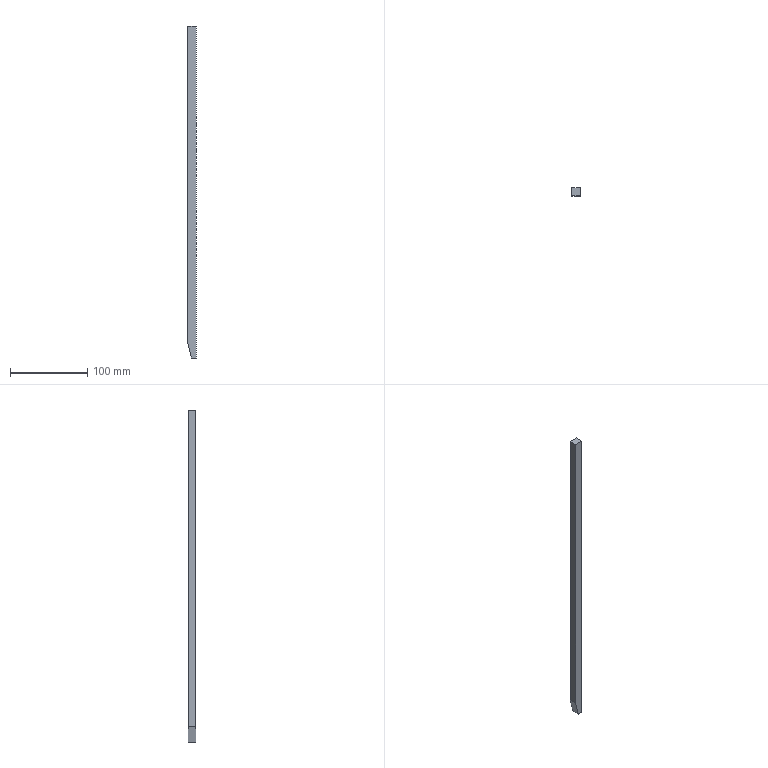Component | SolidWorks | CHEN123-AA-19-1 | 1 solid | 7 faces | box 11.5 x 10 x 430 mm | volume 48950 mm3 | plane 7
build123d program:
from build123d import *

# Parameters (mm, degrees)
SKETCH1_W           = 430
SKETCH1_H           = 11.5
BOSS_EXTRUDE1_DEPTH = 10
CHAMFER1_SIZE       = 20
CHAMFER1_SIZE2      = 5


with BuildPart() as part:
    # Sketch1 → Boss-Extrude1 (new body)
    with BuildSketch(Plane.XY):
        Rectangle(SKETCH1_W, SKETCH1_H)
    extrude(amount=BOSS_EXTRUDE1_DEPTH)

    # Chamfer1
    chamfer1_edges = [part.edges().sort_by_distance(p)[0] for p in [
        (-215, -5.75, 5),
    ]]
    chamfer1_side = [part.faces().sort_by_distance(p)[0] for p in [
        (0, -5.75, 5),
    ]]
    chamfer(chamfer1_edges, length=CHAMFER1_SIZE, length2=CHAMFER1_SIZE2, reference=chamfer1_side[0])


solid = part.part

# Placed as in the assembly
solid = solid.moved(Location((22.25, 34.001, -205), (-90, 0, -90)))
STEP:
#1=COLOUR_RGB('',0.7922,0.8196,0.9333);
#2=FILL_AREA_STYLE_COLOUR('',#1);
#3=FILL_AREA_STYLE('',(#2));
#4=SURFACE_STYLE_FILL_AREA(#3);
#5=SURFACE_SIDE_STYLE('',(#4));
#6=SURFACE_STYLE_USAGE(.BOTH.,#5);
#7=PRESENTATION_STYLE_ASSIGNMENT((#6));
#8=CARTESIAN_POINT('',(0.6496,1.339,0.3937));
#9=VERTEX_POINT('',#8);
#10=CARTESIAN_POINT('',(1.102,1.339,0.3937));
#11=VERTEX_POINT('',#10);
#12=CARTESIAN_POINT('',(0.6496,1.339,0.3937));
#13=DIRECTION('',(1.,-0.,-0.));
#14=VECTOR('',#13,39.37);
#15=LINE('',#12,#14);
#16=EDGE_CURVE('',#9,#11,#15,.T.);
#17=ORIENTED_EDGE('',*,*,#16,.T.);
#18=CARTESIAN_POINT('',(1.102,1.732,0.3937));
#19=VERTEX_POINT('',#18);
#20=CARTESIAN_POINT('',(1.102,1.732,0.3937));
#21=DIRECTION('',(-0.,-1.,0.));
#22=VECTOR('',#21,39.37);
#23=LINE('',#20,#22);
#24=EDGE_CURVE('',#19,#11,#23,.T.);
#25=ORIENTED_EDGE('',*,*,#24,.F.);
#26=CARTESIAN_POINT('',(0.6496,1.732,0.3937));
#27=VERTEX_POINT('',#26);
#28=CARTESIAN_POINT('',(0.6496,1.732,0.3937));
#29=DIRECTION('',(1.,-0.,-0.));
#30=VECTOR('',#29,39.37);
#31=LINE('',#28,#30);
#32=EDGE_CURVE('',#27,#19,#31,.T.);
#33=ORIENTED_EDGE('',*,*,#32,.F.);
#34=CARTESIAN_POINT('',(0.6496,1.732,0.3937));
#35=DIRECTION('',(-0.,-1.,0.));
#36=VECTOR('',#35,39.37);
#37=LINE('',#34,#36);
#38=EDGE_CURVE('',#27,#9,#37,.T.);
#39=ORIENTED_EDGE('',*,*,#38,.T.);
#40=EDGE_LOOP('',(#17,#25,#33,#39));
#41=FACE_OUTER_BOUND('',#40,.T.);
#42=CARTESIAN_POINT('',(0.6496,1.732,0.3937));
#43=DIRECTION('',(-0.,-0.,-1.));
#44=DIRECTION('',(0.,1.,-0.));
#45=AXIS2_PLACEMENT_3D('',#42,#43,#44);
#46=PLANE('',#45);
#47=ADVANCED_FACE('',(#41),#46,.F.);
#48=CARTESIAN_POINT('',(1.102,1.339,-16.535));
#49=VERTEX_POINT('',#48);
#50=CARTESIAN_POINT('',(1.102,1.339,-16.535));
#51=DIRECTION('',(-0.,0.,-1.));
#52=VECTOR('',#51,39.37);
#53=LINE('',#50,#52);
#54=EDGE_CURVE('',#11,#49,#53,.T.);
#55=ORIENTED_EDGE('',*,*,#54,.T.);
#56=CARTESIAN_POINT('',(1.102,1.732,-16.535));
#57=VERTEX_POINT('',#56);
#58=CARTESIAN_POINT('',(1.102,1.732,-16.535));
#59=DIRECTION('',(-0.,-1.,0.));
#60=VECTOR('',#59,39.37);
#61=LINE('',#58,#60);
#62=EDGE_CURVE('',#57,#49,#61,.T.);
#63=ORIENTED_EDGE('',*,*,#62,.F.);
#64=CARTESIAN_POINT('',(1.102,1.732,-16.535));
#65=DIRECTION('',(-0.,0.,-1.));
#66=VECTOR('',#65,39.37);
#67=LINE('',#64,#66);
#68=EDGE_CURVE('',#19,#57,#67,.T.);
#69=ORIENTED_EDGE('',*,*,#68,.F.);
#70=ORIENTED_EDGE('',*,*,#24,.T.);
#71=EDGE_LOOP('',(#55,#63,#69,#70));
#72=FACE_OUTER_BOUND('',#71,.T.);
#73=CARTESIAN_POINT('',(1.102,1.732,-16.535));
#74=DIRECTION('',(-1.,0.,0.));
#75=DIRECTION('',(-0.,-1.,0.));
#76=AXIS2_PLACEMENT_3D('',#73,#74,#75);
#77=PLANE('',#76);
#78=ADVANCED_FACE('',(#72),#77,.F.);
#79=CARTESIAN_POINT('',(0.8464,1.339,-16.535));
#80=VERTEX_POINT('',#79);
#81=CARTESIAN_POINT('',(0.6496,1.339,-16.535));
#82=DIRECTION('',(-1.,0.,0.));
#83=VECTOR('',#82,39.37);
#84=LINE('',#81,#83);
#85=EDGE_CURVE('',#49,#80,#84,.T.);
#86=ORIENTED_EDGE('',*,*,#85,.T.);
#87=CARTESIAN_POINT('',(0.8464,1.732,-16.535));
#88=VERTEX_POINT('',#87);
#89=CARTESIAN_POINT('',(0.8464,1.732,-16.535));
#90=DIRECTION('',(0.,1.,-0.));
#91=VECTOR('',#90,39.37);
#92=LINE('',#89,#91);
#93=EDGE_CURVE('',#80,#88,#92,.T.);
#94=ORIENTED_EDGE('',*,*,#93,.T.);
#95=CARTESIAN_POINT('',(0.6496,1.732,-16.535));
#96=DIRECTION('',(-1.,0.,0.));
#97=VECTOR('',#96,39.37);
#98=LINE('',#95,#97);
#99=EDGE_CURVE('',#57,#88,#98,.T.);
#100=ORIENTED_EDGE('',*,*,#99,.F.);
#101=ORIENTED_EDGE('',*,*,#62,.T.);
#102=EDGE_LOOP('',(#86,#94,#100,#101));
#103=FACE_OUTER_BOUND('',#102,.T.);
#104=CARTESIAN_POINT('',(0.6496,1.732,-16.535));
#105=DIRECTION('',(0.,0.,1.));
#106=DIRECTION('',(-0.,-1.,0.));
#107=AXIS2_PLACEMENT_3D('',#104,#105,#106);
#108=PLANE('',#107);
#109=ADVANCED_FACE('',(#103),#108,.F.);
#110=CARTESIAN_POINT('',(0.6496,1.732,-15.748));
#111=VERTEX_POINT('',#110);
#112=CARTESIAN_POINT('',(0.6496,1.732,-16.535));
#113=DIRECTION('',(0.,-0.,1.));
#114=VECTOR('',#113,39.37);
#115=LINE('',#112,#114);
#116=EDGE_CURVE('',#111,#27,#115,.T.);
#117=ORIENTED_EDGE('',*,*,#116,.F.);
#118=CARTESIAN_POINT('',(0.6496,1.339,-15.748));
#119=VERTEX_POINT('',#118);
#120=CARTESIAN_POINT('',(0.6496,1.732,-15.748));
#121=DIRECTION('',(-0.,-1.,0.));
#122=VECTOR('',#121,39.37);
#123=LINE('',#120,#122);
#124=EDGE_CURVE('',#111,#119,#123,.T.);
#125=ORIENTED_EDGE('',*,*,#124,.T.);
#126=CARTESIAN_POINT('',(0.6496,1.339,-16.535));
#127=DIRECTION('',(0.,-0.,1.));
#128=VECTOR('',#127,39.37);
#129=LINE('',#126,#128);
#130=EDGE_CURVE('',#119,#9,#129,.T.);
#131=ORIENTED_EDGE('',*,*,#130,.T.);
#132=ORIENTED_EDGE('',*,*,#38,.F.);
#133=EDGE_LOOP('',(#117,#125,#131,#132));
#134=FACE_OUTER_BOUND('',#133,.T.);
#135=CARTESIAN_POINT('',(0.6496,1.732,-16.535));
#136=DIRECTION('',(1.,-0.,-0.));
#137=DIRECTION('',(0.,1.,-0.));
#138=AXIS2_PLACEMENT_3D('',#135,#136,#137);
#139=PLANE('',#138);
#140=ADVANCED_FACE('',(#134),#139,.F.);
#141=ORIENTED_EDGE('',*,*,#99,.T.);
#142=CARTESIAN_POINT('',(0.6496,1.732,-15.748));
#143=DIRECTION('',(-0.2425,-0.,0.9701));
#144=VECTOR('',#143,39.37);
#145=LINE('',#142,#144);
#146=EDGE_CURVE('',#88,#111,#145,.T.);
#147=ORIENTED_EDGE('',*,*,#146,.T.);
#148=ORIENTED_EDGE('',*,*,#116,.T.);
#149=ORIENTED_EDGE('',*,*,#32,.T.);
#150=ORIENTED_EDGE('',*,*,#68,.T.);
#151=EDGE_LOOP('',(#141,#147,#148,#149,#150));
#152=FACE_OUTER_BOUND('',#151,.T.);
#153=CARTESIAN_POINT('',(0.876,1.732,-8.071));
#154=DIRECTION('',(-0.,-1.,-0.));
#155=DIRECTION('',(-0.,0.,-1.));
#156=AXIS2_PLACEMENT_3D('',#153,#154,#155);
#157=PLANE('',#156);
#158=ADVANCED_FACE('',(#152),#157,.F.);
#159=ORIENTED_EDGE('',*,*,#130,.F.);
#160=CARTESIAN_POINT('',(-1.143,1.339,-8.576));
#161=DIRECTION('',(0.2425,0.,-0.9701));
#162=VECTOR('',#161,39.37);
#163=LINE('',#160,#162);
#164=EDGE_CURVE('',#119,#80,#163,.T.);
#165=ORIENTED_EDGE('',*,*,#164,.T.);
#166=ORIENTED_EDGE('',*,*,#85,.F.);
#167=ORIENTED_EDGE('',*,*,#54,.F.);
#168=ORIENTED_EDGE('',*,*,#16,.F.);
#169=EDGE_LOOP('',(#159,#165,#166,#167,#168));
#170=FACE_OUTER_BOUND('',#169,.T.);
#171=CARTESIAN_POINT('',(0.876,1.339,-8.071));
#172=DIRECTION('',(-0.,-1.,-0.));
#173=DIRECTION('',(-0.,0.,-1.));
#174=AXIS2_PLACEMENT_3D('',#171,#172,#173);
#175=PLANE('',#174);
#176=ADVANCED_FACE('',(#170),#175,.T.);
#177=ORIENTED_EDGE('',*,*,#146,.F.);
#178=ORIENTED_EDGE('',*,*,#93,.F.);
#179=ORIENTED_EDGE('',*,*,#164,.F.);
#180=ORIENTED_EDGE('',*,*,#124,.F.);
#181=EDGE_LOOP('',(#177,#178,#179,#180));
#182=FACE_OUTER_BOUND('',#181,.T.);
#183=CARTESIAN_POINT('',(0.6496,1.732,-15.748));
#184=DIRECTION('',(0.9701,0.,0.2425));
#185=DIRECTION('',(-0.,-1.,0.));
#186=AXIS2_PLACEMENT_3D('',#183,#184,#185);
#187=PLANE('',#186);
#188=ADVANCED_FACE('',(#182),#187,.F.);
#189=CLOSED_SHELL('',(#47,#78,#109,#140,#158,#176,#188));
#190=MANIFOLD_SOLID_BREP('',#189);
#191=STYLED_ITEM('',(#7),#190);
#192=(LENGTH_UNIT()NAMED_UNIT(*)SI_UNIT($,.METRE.));
#193=LENGTH_MEASURE_WITH_UNIT(LENGTH_MEASURE(0.0254),#192);
#194=DIMENSIONAL_EXPONENTS(1.,0.,0.,0.,0.,0.,0.);
#195=(CONVERSION_BASED_UNIT('',#193)LENGTH_UNIT()NAMED_UNIT(#194));
#196=UNCERTAINTY_MEASURE_WITH_UNIT(LENGTH_MEASURE(0.00001),#195,'','');
#197=(NAMED_UNIT(*)PLANE_ANGLE_UNIT()SI_UNIT($,.RADIAN.));
#198=(NAMED_UNIT(*)SI_UNIT($,.STERADIAN.)SOLID_ANGLE_UNIT());
#199=(GEOMETRIC_REPRESENTATION_CONTEXT(3)GLOBAL_UNCERTAINTY_ASSIGNED_CONTEXT((#196))GLOBAL_UNIT_ASSIGNED_CONTEXT((#195,#197,#198))REPRESENTATION_CONTEXT('',''));
#200=MECHANICAL_DESIGN_GEOMETRIC_PRESENTATION_REPRESENTATION('',(#191),#199);
#201=CARTESIAN_POINT('',(0.,0.,0.));
#202=DIRECTION('',(0.,0.,1.));
#203=DIRECTION('',(1.,0.,0.));
#204=AXIS2_PLACEMENT_3D('',#201,#202,#203);
#205=(LENGTH_UNIT()NAMED_UNIT(*)SI_UNIT($,.METRE.));
#206=LENGTH_MEASURE_WITH_UNIT(LENGTH_MEASURE(0.0254),#205);
#207=DIMENSIONAL_EXPONENTS(1.,0.,0.,0.,0.,0.,0.);
#208=(CONVERSION_BASED_UNIT('',#206)LENGTH_UNIT()NAMED_UNIT(#207));
#209=UNCERTAINTY_MEASURE_WITH_UNIT(LENGTH_MEASURE(0.00001),#208,'','');
#210=(NAMED_UNIT(*)PLANE_ANGLE_UNIT()SI_UNIT($,.RADIAN.));
#211=(NAMED_UNIT(*)SI_UNIT($,.STERADIAN.)SOLID_ANGLE_UNIT());
#212=(GEOMETRIC_REPRESENTATION_CONTEXT(3)GLOBAL_UNCERTAINTY_ASSIGNED_CONTEXT((#209))GLOBAL_UNIT_ASSIGNED_CONTEXT((#208,#210,#211))REPRESENTATION_CONTEXT('',''));
#213=ADVANCED_BREP_SHAPE_REPRESENTATION('',(#190,#204),#212);
#214=PRESENTATION_LAYER_ASSIGNMENT('','',(#191));